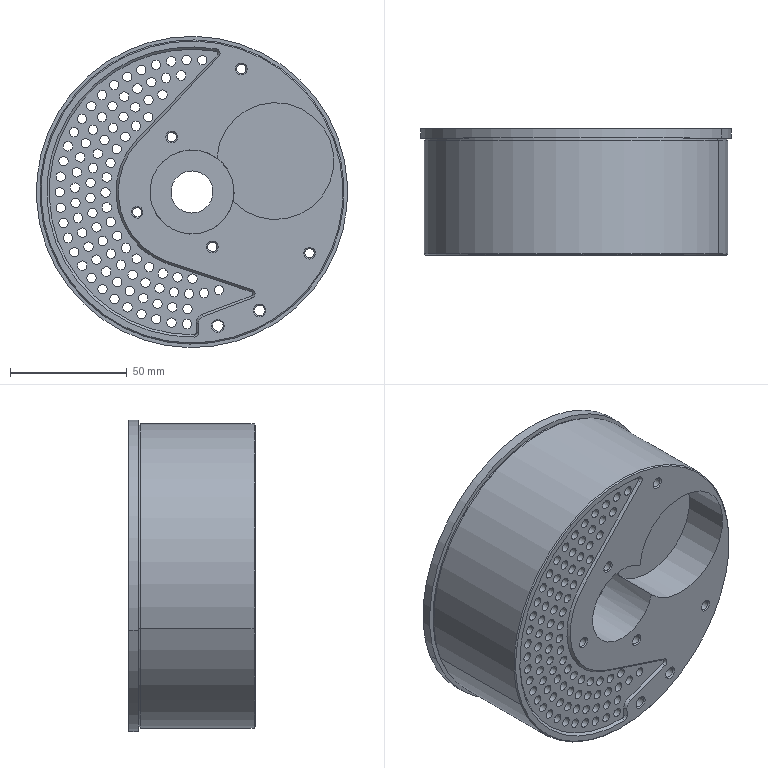Component | SolidWorks | Gearbox Housing-1 | 1 solid | 270 faces | box 133 x 54 x 133 mm | volume 172727 mm3 | cylinder 223 | cone 25 | plane 20 | torus 2 | commonest cylinder face diameters 4 x190 4.5 x4 2 x4 48 x4 129 x2 36 x2 23 x2 35 x2